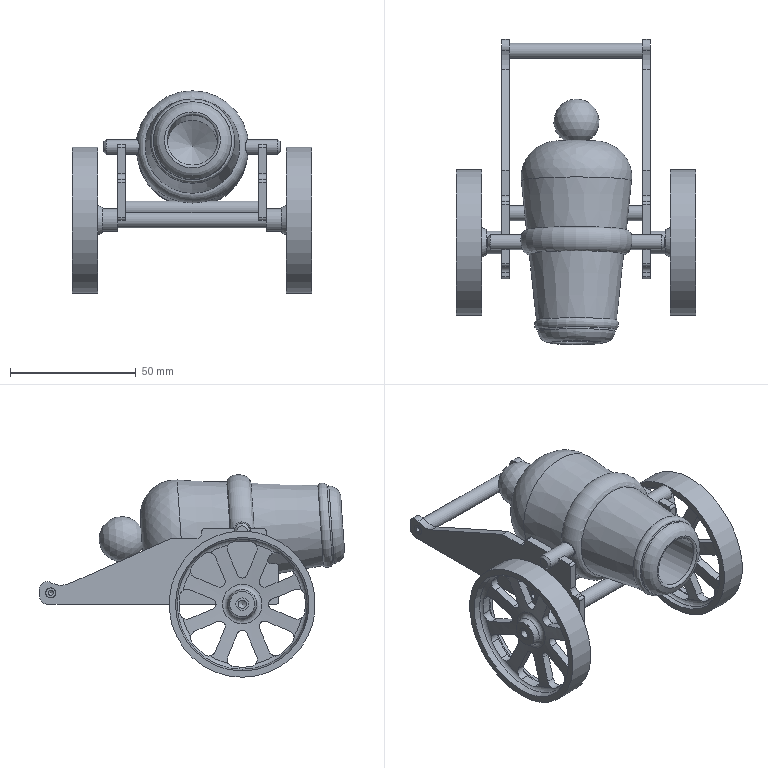Assembly | NX | mm | 12 component files | 12 solids | 251 faces | box 95 x 121.13 x 80.72 mm | volume 120368 mm3 | cylinder 118 | plane 90 | cone 27 | torus 10 | spline 3 | other 2 | sphere 1 | commonest cylinder face diameters 5.6 x32 50 x16 4.2 x16 2 x12 6 x9 5 x8 6.2 x4 4 x4
Bill of materials:
unnamed part 1 | 2 |  | Spoked wheel: a flat cylindrical rim with eight straight radial spokes joining a central hub that has a small center bore. The hub sticks out from one face.
unnamed part 2 | 1 |  | Hollow, roughly bottle- or knob-shaped body of revolution. One end is a closed dome and the body tapers toward the other end, which is open. There is a raised ring band near the middle with a small radial cross hole, and a textured bead ring near the open end.
unnamed part 3 | 2 |  | Long straight cylindrical rod with a short, smaller-diameter stepped section at each end. There is a small central recess or bore in the end face.
unnamed part 4 | 1 |  | Ball-shaped knob: a sphere with a solid cylindrical stem sticking out on one side. The stem end has a chamfer.
unnamed part 5 | 1 |  | Plain straight solid cylindrical pin or rod with small chamfers at both ends.
unnamed part 6 | 2 |  | Plain cylindrical tube or sleeve with a concentric through bore. The ends are flat and square.
unnamed part 7 | 2 |  | Flat plate bracket with a tapered profile and constant thickness. One end is wider and has semicircular edge notches and stepped corners. The plate narrows to a rounded lug at the other end, which has a round hole. A second round hole sits near the wide end.
unnamed part 8 | 1 |  | Long cylindrical shaft with longer reduced-diameter stepped sections at both ends. The end face shows a central bore or recess.
Mates:
1. bond | bracket 2 component | assembly component
2. bond | bracket 2 component | assembly component
3. bond | bracket 1 component | assembly component
4. linear | assembly datumaxis | assembly cartesiancoordinatesystem | assembly cartesiancoordinatesystem
5. fix | bracket 2 component
6. touch align | support 1 face | bracket 2 face
7. center | support 1 face | support 1 face | bracket 1 face | bracket 2 face
8. touch align | barrel 1 face | support 1 face
9. concentric | plug 1 edge | barrel 1 edge
10. concentric | shaft 2 edge | bracket 2 edge
11. concentric | bushing 2 edge | wheel_axle 1 edge
12. concentric | bushing 2 edge | bracket 1 edge
13. concentric | bushing 1 edge | bracket 2 edge
14. concentric | wheel 2 edge | bushing 2 edge
15. concentric | wheel 1 edge | bushing 1 edge
16. concentric | shaft 1 edge | bracket 2 edge